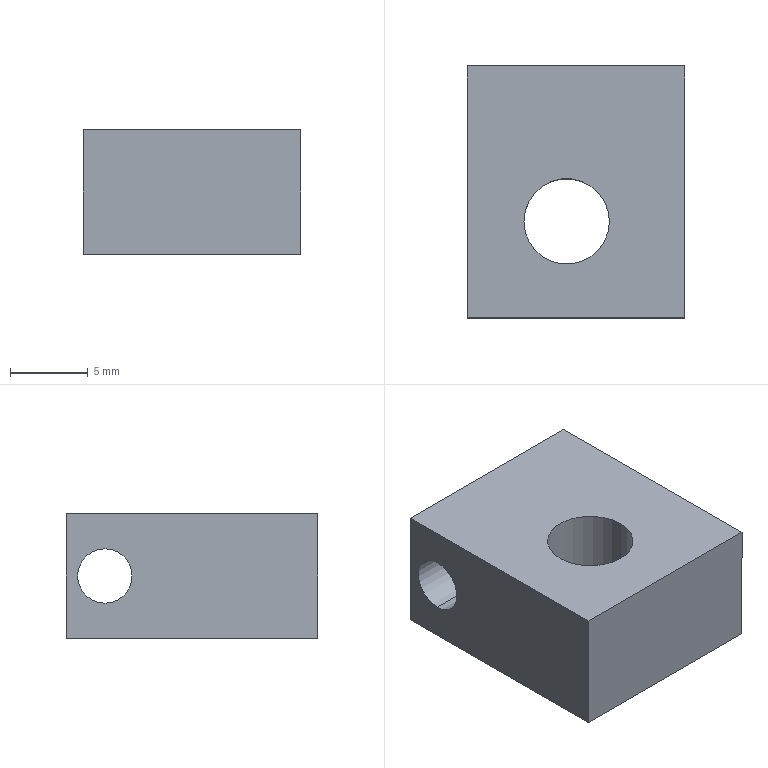Component | SolidWorks | PointedHeadInspectionPart-2 | 1 solid | 10 faces | box 14 x 16.2 x 8 mm | volume 1490 mm3 | plane 6 | cylinder 4 | commonest cylinder face diameters 5.5 x2 3.5 x2
build123d program:
from build123d import *

# Parameters (mm, degrees)
SKETCH1_W          = 14
SKETCH1_H          = 8
EXTRUDE1_DEPTH     = 16.2
SKETCH2_R          = 1.75
CUT_EXTRUDE1_DEPTH = 23.857
SKETCH3_R          = 2.75
CUT_EXTRUDE2_DEPTH = 23.857


with BuildPart() as part:
    # Sketch1 → Extrude1 (new body)
    with BuildSketch(Plane(origin=(0, 0, 0), x_dir=(1, 0, 0), z_dir=(0, 1, 0))):
        with Locations((7, -4)):
            Rectangle(SKETCH1_W, SKETCH1_H)
    extrude(amount=EXTRUDE1_DEPTH)

    # Sketch2 → Cut-Extrude1 (cut, through all)
    with BuildSketch(Plane(origin=(14, 0, 0), x_dir=(0, 0, -1), z_dir=(1, 0, 0))):
        with Locations((-4, 13.7)):
            Circle(SKETCH2_R)
    extrude(amount=-CUT_EXTRUDE1_DEPTH, mode=Mode.SUBTRACT)

    # Sketch3 → Cut-Extrude2 (cut, through all)
    with BuildSketch(Plane.XY.offset(8)):
        with Locations((6.4, 6.2)):
            Circle(SKETCH3_R)
    extrude(amount=-CUT_EXTRUDE2_DEPTH, mode=Mode.SUBTRACT)


solid = part.part

# Placed as in the assembly
solid = solid.moved(Location((25.617, 66.172, -56.387), (0, 0, 0)))
STEP:
#1=COLOUR_RGB('',0.7922,0.8196,0.9333);
#2=FILL_AREA_STYLE_COLOUR('',#1);
#3=FILL_AREA_STYLE('',(#2));
#4=SURFACE_STYLE_FILL_AREA(#3);
#5=SURFACE_SIDE_STYLE('',(#4));
#6=SURFACE_STYLE_USAGE(.BOTH.,#5);
#7=PRESENTATION_STYLE_ASSIGNMENT((#6));
#8=CARTESIAN_POINT('',(1.152,2.849,-2.22));
#9=VERTEX_POINT('',#8);
#10=CARTESIAN_POINT('',(1.369,2.849,-2.22));
#11=VERTEX_POINT('',#10);
#12=CARTESIAN_POINT('',(1.261,2.849,-2.22));
#13=DIRECTION('',(0.,0.,1.));
#14=DIRECTION('',(1.,0.,0.));
#15=AXIS2_PLACEMENT_3D('',#12,#13,#14);
#16=CIRCLE('',#15,0.1083);
#17=EDGE_CURVE('',#9,#11,#16,.T.);
#18=ORIENTED_EDGE('',*,*,#17,.F.);
#19=CARTESIAN_POINT('',(1.152,2.849,-1.905));
#20=VERTEX_POINT('',#19);
#21=CARTESIAN_POINT('',(1.152,2.849,-2.22));
#22=DIRECTION('',(0.,0.,1.));
#23=VECTOR('',#22,39.37);
#24=LINE('',#21,#23);
#25=EDGE_CURVE('',#9,#20,#24,.T.);
#26=ORIENTED_EDGE('',*,*,#25,.T.);
#27=CARTESIAN_POINT('',(1.369,2.849,-1.905));
#28=VERTEX_POINT('',#27);
#29=CARTESIAN_POINT('',(1.261,2.849,-1.905));
#30=DIRECTION('',(0.,0.,1.));
#31=DIRECTION('',(1.,0.,0.));
#32=AXIS2_PLACEMENT_3D('',#29,#30,#31);
#33=CIRCLE('',#32,0.1083);
#34=EDGE_CURVE('',#20,#28,#33,.T.);
#35=ORIENTED_EDGE('',*,*,#34,.T.);
#36=CARTESIAN_POINT('',(1.369,2.849,-2.22));
#37=DIRECTION('',(0.,0.,1.));
#38=VECTOR('',#37,39.37);
#39=LINE('',#36,#38);
#40=EDGE_CURVE('',#11,#28,#39,.T.);
#41=ORIENTED_EDGE('',*,*,#40,.F.);
#42=EDGE_LOOP('',(#18,#26,#35,#41));
#43=FACE_OUTER_BOUND('',#42,.T.);
#44=CARTESIAN_POINT('',(1.261,2.849,-2.22));
#45=DIRECTION('',(0.,0.,1.));
#46=DIRECTION('',(1.,0.,0.));
#47=AXIS2_PLACEMENT_3D('',#44,#45,#46);
#48=CYLINDRICAL_SURFACE('',#47,0.1083);
#49=ADVANCED_FACE('',(#43),#48,.F.);
#50=CARTESIAN_POINT('',(1.009,3.145,-1.994));
#51=VERTEX_POINT('',#50);
#52=CARTESIAN_POINT('',(1.009,3.145,-2.131));
#53=VERTEX_POINT('',#52);
#54=CARTESIAN_POINT('',(1.009,3.145,-2.062));
#55=DIRECTION('',(1.,0.,0.));
#56=DIRECTION('',(0.,0.,-1.));
#57=AXIS2_PLACEMENT_3D('',#54,#55,#56);
#58=CIRCLE('',#57,0.0689);
#59=EDGE_CURVE('',#51,#53,#58,.T.);
#60=ORIENTED_EDGE('',*,*,#59,.F.);
#61=CARTESIAN_POINT('',(1.56,3.145,-1.994));
#62=VERTEX_POINT('',#61);
#63=CARTESIAN_POINT('',(1.009,3.145,-1.994));
#64=DIRECTION('',(1.,0.,0.));
#65=VECTOR('',#64,39.37);
#66=LINE('',#63,#65);
#67=EDGE_CURVE('',#51,#62,#66,.T.);
#68=ORIENTED_EDGE('',*,*,#67,.T.);
#69=CARTESIAN_POINT('',(1.56,3.145,-2.131));
#70=VERTEX_POINT('',#69);
#71=CARTESIAN_POINT('',(1.56,3.145,-2.062));
#72=DIRECTION('',(1.,0.,0.));
#73=DIRECTION('',(0.,0.,-1.));
#74=AXIS2_PLACEMENT_3D('',#71,#72,#73);
#75=CIRCLE('',#74,0.0689);
#76=EDGE_CURVE('',#62,#70,#75,.T.);
#77=ORIENTED_EDGE('',*,*,#76,.T.);
#78=CARTESIAN_POINT('',(1.009,3.145,-2.131));
#79=DIRECTION('',(1.,0.,0.));
#80=VECTOR('',#79,39.37);
#81=LINE('',#78,#80);
#82=EDGE_CURVE('',#53,#70,#81,.T.);
#83=ORIENTED_EDGE('',*,*,#82,.F.);
#84=EDGE_LOOP('',(#60,#68,#77,#83));
#85=FACE_OUTER_BOUND('',#84,.T.);
#86=CARTESIAN_POINT('',(1.009,3.145,-2.062));
#87=DIRECTION('',(1.,0.,0.));
#88=DIRECTION('',(0.,0.,-1.));
#89=AXIS2_PLACEMENT_3D('',#86,#87,#88);
#90=CYLINDRICAL_SURFACE('',#89,0.0689);
#91=ADVANCED_FACE('',(#85),#90,.F.);
#92=CARTESIAN_POINT('',(1.009,3.145,-2.062));
#93=DIRECTION('',(1.,0.,0.));
#94=DIRECTION('',(0.,0.,-1.));
#95=AXIS2_PLACEMENT_3D('',#92,#93,#94);
#96=CIRCLE('',#95,0.0689);
#97=EDGE_CURVE('',#53,#51,#96,.T.);
#98=ORIENTED_EDGE('',*,*,#97,.T.);
#99=ORIENTED_EDGE('',*,*,#59,.T.);
#100=EDGE_LOOP('',(#98,#99));
#101=FACE_BOUND('',#100,.T.);
#102=CARTESIAN_POINT('',(1.009,2.605,-2.22));
#103=VERTEX_POINT('',#102);
#104=CARTESIAN_POINT('',(1.009,2.605,-1.905));
#105=VERTEX_POINT('',#104);
#106=CARTESIAN_POINT('',(1.009,2.605,-2.22));
#107=DIRECTION('',(0.,0.,1.));
#108=VECTOR('',#107,39.37);
#109=LINE('',#106,#108);
#110=EDGE_CURVE('',#103,#105,#109,.T.);
#111=ORIENTED_EDGE('',*,*,#110,.T.);
#112=CARTESIAN_POINT('',(1.009,3.243,-1.905));
#113=VERTEX_POINT('',#112);
#114=CARTESIAN_POINT('',(1.009,3.243,-1.905));
#115=DIRECTION('',(0.,-1.,0.));
#116=VECTOR('',#115,39.37);
#117=LINE('',#114,#116);
#118=EDGE_CURVE('',#113,#105,#117,.T.);
#119=ORIENTED_EDGE('',*,*,#118,.F.);
#120=CARTESIAN_POINT('',(1.009,3.243,-2.22));
#121=VERTEX_POINT('',#120);
#122=CARTESIAN_POINT('',(1.009,3.243,-2.22));
#123=DIRECTION('',(0.,0.,1.));
#124=VECTOR('',#123,39.37);
#125=LINE('',#122,#124);
#126=EDGE_CURVE('',#121,#113,#125,.T.);
#127=ORIENTED_EDGE('',*,*,#126,.F.);
#128=CARTESIAN_POINT('',(1.009,3.243,-2.22));
#129=DIRECTION('',(0.,-1.,0.));
#130=VECTOR('',#129,39.37);
#131=LINE('',#128,#130);
#132=EDGE_CURVE('',#121,#103,#131,.T.);
#133=ORIENTED_EDGE('',*,*,#132,.T.);
#134=EDGE_LOOP('',(#111,#119,#127,#133));
#135=FACE_OUTER_BOUND('',#134,.T.);
#136=CARTESIAN_POINT('',(1.009,3.243,-2.22));
#137=DIRECTION('',(1.,0.,-0.));
#138=DIRECTION('',(-0.,0.,-1.));
#139=AXIS2_PLACEMENT_3D('',#136,#137,#138);
#140=PLANE('',#139);
#141=ADVANCED_FACE('',(#101,#135),#140,.F.);
#142=CARTESIAN_POINT('',(1.261,2.849,-1.905));
#143=DIRECTION('',(0.,0.,1.));
#144=DIRECTION('',(1.,0.,0.));
#145=AXIS2_PLACEMENT_3D('',#142,#143,#144);
#146=CIRCLE('',#145,0.1083);
#147=EDGE_CURVE('',#28,#20,#146,.T.);
#148=ORIENTED_EDGE('',*,*,#147,.F.);
#149=ORIENTED_EDGE('',*,*,#34,.F.);
#150=EDGE_LOOP('',(#148,#149));
#151=FACE_BOUND('',#150,.T.);
#152=CARTESIAN_POINT('',(1.56,2.605,-1.905));
#153=VERTEX_POINT('',#152);
#154=CARTESIAN_POINT('',(1.009,2.605,-1.905));
#155=DIRECTION('',(1.,0.,0.));
#156=VECTOR('',#155,39.37);
#157=LINE('',#154,#156);
#158=EDGE_CURVE('',#105,#153,#157,.T.);
#159=ORIENTED_EDGE('',*,*,#158,.T.);
#160=CARTESIAN_POINT('',(1.56,3.243,-1.905));
#161=VERTEX_POINT('',#160);
#162=CARTESIAN_POINT('',(1.56,3.243,-1.905));
#163=DIRECTION('',(0.,-1.,0.));
#164=VECTOR('',#163,39.37);
#165=LINE('',#162,#164);
#166=EDGE_CURVE('',#161,#153,#165,.T.);
#167=ORIENTED_EDGE('',*,*,#166,.F.);
#168=CARTESIAN_POINT('',(1.009,3.243,-1.905));
#169=DIRECTION('',(1.,0.,0.));
#170=VECTOR('',#169,39.37);
#171=LINE('',#168,#170);
#172=EDGE_CURVE('',#113,#161,#171,.T.);
#173=ORIENTED_EDGE('',*,*,#172,.F.);
#174=ORIENTED_EDGE('',*,*,#118,.T.);
#175=EDGE_LOOP('',(#159,#167,#173,#174));
#176=FACE_OUTER_BOUND('',#175,.T.);
#177=CARTESIAN_POINT('',(1.009,3.243,-1.905));
#178=DIRECTION('',(0.,0.,-1.));
#179=DIRECTION('',(-1.,0.,0.));
#180=AXIS2_PLACEMENT_3D('',#177,#178,#179);
#181=PLANE('',#180);
#182=ADVANCED_FACE('',(#151,#176),#181,.F.);
#183=CARTESIAN_POINT('',(1.56,3.145,-2.062));
#184=DIRECTION('',(1.,0.,0.));
#185=DIRECTION('',(0.,0.,-1.));
#186=AXIS2_PLACEMENT_3D('',#183,#184,#185);
#187=CIRCLE('',#186,0.0689);
#188=EDGE_CURVE('',#70,#62,#187,.T.);
#189=ORIENTED_EDGE('',*,*,#188,.F.);
#190=ORIENTED_EDGE('',*,*,#76,.F.);
#191=EDGE_LOOP('',(#189,#190));
#192=FACE_BOUND('',#191,.T.);
#193=CARTESIAN_POINT('',(1.56,2.605,-2.22));
#194=VERTEX_POINT('',#193);
#195=CARTESIAN_POINT('',(1.56,2.605,-2.22));
#196=DIRECTION('',(-0.,0.,-1.));
#197=VECTOR('',#196,39.37);
#198=LINE('',#195,#197);
#199=EDGE_CURVE('',#153,#194,#198,.T.);
#200=ORIENTED_EDGE('',*,*,#199,.T.);
#201=CARTESIAN_POINT('',(1.56,3.243,-2.22));
#202=VERTEX_POINT('',#201);
#203=CARTESIAN_POINT('',(1.56,3.243,-2.22));
#204=DIRECTION('',(0.,-1.,0.));
#205=VECTOR('',#204,39.37);
#206=LINE('',#203,#205);
#207=EDGE_CURVE('',#202,#194,#206,.T.);
#208=ORIENTED_EDGE('',*,*,#207,.F.);
#209=CARTESIAN_POINT('',(1.56,3.243,-2.22));
#210=DIRECTION('',(-0.,0.,-1.));
#211=VECTOR('',#210,39.37);
#212=LINE('',#209,#211);
#213=EDGE_CURVE('',#161,#202,#212,.T.);
#214=ORIENTED_EDGE('',*,*,#213,.F.);
#215=ORIENTED_EDGE('',*,*,#166,.T.);
#216=EDGE_LOOP('',(#200,#208,#214,#215));
#217=FACE_OUTER_BOUND('',#216,.T.);
#218=CARTESIAN_POINT('',(1.56,3.243,-2.22));
#219=DIRECTION('',(-1.,0.,0.));
#220=DIRECTION('',(0.,0.,1.));
#221=AXIS2_PLACEMENT_3D('',#218,#219,#220);
#222=PLANE('',#221);
#223=ADVANCED_FACE('',(#192,#217),#222,.F.);
#224=CARTESIAN_POINT('',(1.261,2.849,-2.22));
#225=DIRECTION('',(0.,0.,1.));
#226=DIRECTION('',(1.,0.,0.));
#227=AXIS2_PLACEMENT_3D('',#224,#225,#226);
#228=CIRCLE('',#227,0.1083);
#229=EDGE_CURVE('',#11,#9,#228,.T.);
#230=ORIENTED_EDGE('',*,*,#229,.T.);
#231=ORIENTED_EDGE('',*,*,#17,.T.);
#232=EDGE_LOOP('',(#230,#231));
#233=FACE_BOUND('',#232,.T.);
#234=CARTESIAN_POINT('',(1.009,2.605,-2.22));
#235=DIRECTION('',(-1.,0.,0.));
#236=VECTOR('',#235,39.37);
#237=LINE('',#234,#236);
#238=EDGE_CURVE('',#194,#103,#237,.T.);
#239=ORIENTED_EDGE('',*,*,#238,.T.);
#240=ORIENTED_EDGE('',*,*,#132,.F.);
#241=CARTESIAN_POINT('',(1.009,3.243,-2.22));
#242=DIRECTION('',(-1.,0.,0.));
#243=VECTOR('',#242,39.37);
#244=LINE('',#241,#243);
#245=EDGE_CURVE('',#202,#121,#244,.T.);
#246=ORIENTED_EDGE('',*,*,#245,.F.);
#247=ORIENTED_EDGE('',*,*,#207,.T.);
#248=EDGE_LOOP('',(#239,#240,#246,#247));
#249=FACE_OUTER_BOUND('',#248,.T.);
#250=CARTESIAN_POINT('',(1.009,3.243,-2.22));
#251=DIRECTION('',(0.,0.,1.));
#252=DIRECTION('',(1.,0.,0.));
#253=AXIS2_PLACEMENT_3D('',#250,#251,#252);
#254=PLANE('',#253);
#255=ADVANCED_FACE('',(#233,#249),#254,.F.);
#256=ORIENTED_EDGE('',*,*,#126,.T.);
#257=ORIENTED_EDGE('',*,*,#172,.T.);
#258=ORIENTED_EDGE('',*,*,#213,.T.);
#259=ORIENTED_EDGE('',*,*,#245,.T.);
#260=EDGE_LOOP('',(#256,#257,#258,#259));
#261=FACE_OUTER_BOUND('',#260,.T.);
#262=CARTESIAN_POINT('',(1.009,3.243,-1.905));
#263=DIRECTION('',(0.,1.,0.));
#264=DIRECTION('',(0.,0.,1.));
#265=AXIS2_PLACEMENT_3D('',#262,#263,#264);
#266=PLANE('',#265);
#267=ADVANCED_FACE('',(#261),#266,.T.);
#268=ORIENTED_EDGE('',*,*,#110,.F.);
#269=ORIENTED_EDGE('',*,*,#238,.F.);
#270=ORIENTED_EDGE('',*,*,#199,.F.);
#271=ORIENTED_EDGE('',*,*,#158,.F.);
#272=EDGE_LOOP('',(#268,#269,#270,#271));
#273=FACE_OUTER_BOUND('',#272,.T.);
#274=CARTESIAN_POINT('',(1.009,2.605,-1.905));
#275=DIRECTION('',(0.,1.,0.));
#276=DIRECTION('',(0.,0.,1.));
#277=AXIS2_PLACEMENT_3D('',#274,#275,#276);
#278=PLANE('',#277);
#279=ADVANCED_FACE('',(#273),#278,.F.);
#280=ORIENTED_EDGE('',*,*,#67,.F.);
#281=ORIENTED_EDGE('',*,*,#97,.F.);
#282=ORIENTED_EDGE('',*,*,#82,.T.);
#283=ORIENTED_EDGE('',*,*,#188,.T.);
#284=EDGE_LOOP('',(#280,#281,#282,#283));
#285=FACE_OUTER_BOUND('',#284,.T.);
#286=CARTESIAN_POINT('',(1.009,3.145,-2.062));
#287=DIRECTION('',(1.,0.,0.));
#288=DIRECTION('',(0.,0.,-1.));
#289=AXIS2_PLACEMENT_3D('',#286,#287,#288);
#290=CYLINDRICAL_SURFACE('',#289,0.0689);
#291=ADVANCED_FACE('',(#285),#290,.F.);
#292=ORIENTED_EDGE('',*,*,#25,.F.);
#293=ORIENTED_EDGE('',*,*,#229,.F.);
#294=ORIENTED_EDGE('',*,*,#40,.T.);
#295=ORIENTED_EDGE('',*,*,#147,.T.);
#296=EDGE_LOOP('',(#292,#293,#294,#295));
#297=FACE_OUTER_BOUND('',#296,.T.);
#298=CARTESIAN_POINT('',(1.261,2.849,-2.22));
#299=DIRECTION('',(0.,0.,1.));
#300=DIRECTION('',(1.,0.,0.));
#301=AXIS2_PLACEMENT_3D('',#298,#299,#300);
#302=CYLINDRICAL_SURFACE('',#301,0.1083);
#303=ADVANCED_FACE('',(#297),#302,.F.);
#304=CLOSED_SHELL('',(#49,#91,#141,#182,#223,#255,#267,#279,#291,#303));
#305=MANIFOLD_SOLID_BREP('',#304);
#306=STYLED_ITEM('',(#7),#305);
#307=(LENGTH_UNIT()NAMED_UNIT(*)SI_UNIT($,.METRE.));
#308=LENGTH_MEASURE_WITH_UNIT(LENGTH_MEASURE(0.0254),#307);
#309=DIMENSIONAL_EXPONENTS(1.,0.,0.,0.,0.,0.,0.);
#310=(CONVERSION_BASED_UNIT('',#308)LENGTH_UNIT()NAMED_UNIT(#309));
#311=UNCERTAINTY_MEASURE_WITH_UNIT(LENGTH_MEASURE(0.00001),#310,'','');
#312=(NAMED_UNIT(*)PLANE_ANGLE_UNIT()SI_UNIT($,.RADIAN.));
#313=(NAMED_UNIT(*)SI_UNIT($,.STERADIAN.)SOLID_ANGLE_UNIT());
#314=(GEOMETRIC_REPRESENTATION_CONTEXT(3)GLOBAL_UNCERTAINTY_ASSIGNED_CONTEXT((#311))GLOBAL_UNIT_ASSIGNED_CONTEXT((#310,#312,#313))REPRESENTATION_CONTEXT('',''));
#315=MECHANICAL_DESIGN_GEOMETRIC_PRESENTATION_REPRESENTATION('',(#306),#314);
#316=PRESENTATION_LAYER_ASSIGNMENT('','',(#306));
#317=CARTESIAN_POINT('',(0.,0.,0.));
#318=DIRECTION('',(0.,0.,1.));
#319=DIRECTION('',(1.,0.,0.));
#320=AXIS2_PLACEMENT_3D('',#317,#318,#319);
#321=(LENGTH_UNIT()NAMED_UNIT(*)SI_UNIT($,.METRE.));
#322=LENGTH_MEASURE_WITH_UNIT(LENGTH_MEASURE(0.0254),#321);
#323=DIMENSIONAL_EXPONENTS(1.,0.,0.,0.,0.,0.,0.);
#324=(CONVERSION_BASED_UNIT('',#322)LENGTH_UNIT()NAMED_UNIT(#323));
#325=UNCERTAINTY_MEASURE_WITH_UNIT(LENGTH_MEASURE(0.00001),#324,'','');
#326=(NAMED_UNIT(*)PLANE_ANGLE_UNIT()SI_UNIT($,.RADIAN.));
#327=(NAMED_UNIT(*)SI_UNIT($,.STERADIAN.)SOLID_ANGLE_UNIT());
#328=(GEOMETRIC_REPRESENTATION_CONTEXT(3)GLOBAL_UNCERTAINTY_ASSIGNED_CONTEXT((#325))GLOBAL_UNIT_ASSIGNED_CONTEXT((#324,#326,#327))REPRESENTATION_CONTEXT('',''));
#329=ADVANCED_BREP_SHAPE_REPRESENTATION('',(#305,#320),#328);